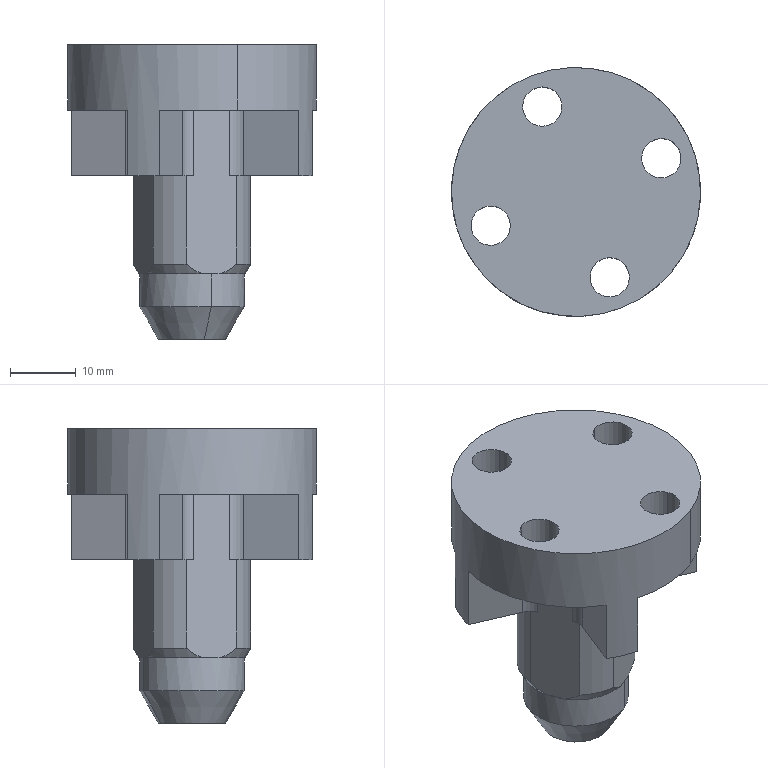Component | SolidWorks | KLHFH005_18LocatingPin-Copy-1 | 1 solid | 56 faces | volume 19866 mm3 | plane 26 | cylinder 24 | cone 6 | commonest cylinder face diameters 6 x16 18 x4 38 x2 16 x2 | material AISI Type A2 Tool Steel